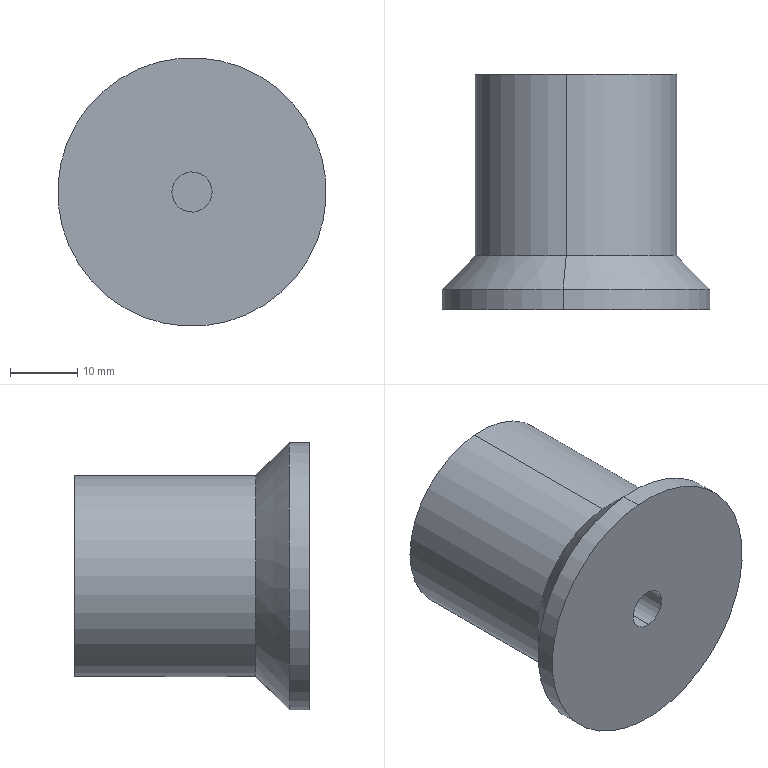Component | SolidWorks | AdjustmentWheel-1 | 1 solid | 13 faces | box 40 x 35 x 40 mm | volume 26932 mm3 | cylinder 8 | plane 3 | cone 2 | commonest cylinder face diameters 2.5 x2 6 x2 40 x2 30 x2
build123d program:
from build123d import *

# Parameters (mm, degrees)
SKETCH2_R      = 3
EXTRUDE2_DEPTH = 25


with BuildPart() as part:
    # Sketch1 → Revolve1 (revolve)
    with BuildSketch(Plane.XY, mode=Mode.PRIVATE) as revolve1_sk:
        Polygon((0, 27.517), (15, 27.517), (15, 0.517), (20, -4.483), (20, -7.483), (0, -7.483), align=None)
    revolve(revolve1_sk.sketch.rotate(Axis((0, 0, 0), (0, 1, 0)), 90), axis=Axis((0, 0, 0), (0, 1, 0)))

    # Sketch2 → Extrude2 (cut)
    with BuildSketch(Plane.XZ.offset(7.483)):
        with Locations(Location((0, 0, 0), (0, 0, 270))):
            Circle(SKETCH2_R)
    extrude(amount=-EXTRUDE2_DEPTH, mode=Mode.SUBTRACT)

    # Sketch3 → M3 Tapped Hole1 (revolve, cut)
    with BuildSketch(Plane(origin=(0, 7.517, 0), x_dir=(0, 1, 0), z_dir=(1, 0, 0))):
        Polygon((0, 0), (0, 20.751), (1.25, 20), (1.25, 0), align=None)
    revolve(axis=Axis((0, 7.517, -6.35), (0, 0, 1)), mode=Mode.SUBTRACT)


solid = part.part

# Placed as in the assembly
solid = solid.moved(Location((-214.784, 725.466, -80.5), (-180, 5.539, 180)))
STEP:
#1=CARTESIAN_POINT('',(-8.399,28.808,-3.757));
#2=VERTEX_POINT('',#1);
#3=CARTESIAN_POINT('',(-8.448,28.858,-3.76));
#4=VERTEX_POINT('',#3);
#5=CARTESIAN_POINT('',(-8.399,28.808,-3.757));
#6=CARTESIAN_POINT('',(-8.405,28.808,-3.758));
#7=CARTESIAN_POINT('',(-8.412,28.81,-3.758));
#8=CARTESIAN_POINT('',(-8.424,28.815,-3.759));
#9=CARTESIAN_POINT('',(-8.429,28.818,-3.759));
#10=CARTESIAN_POINT('',(-8.438,28.827,-3.76));
#11=CARTESIAN_POINT('',(-8.442,28.833,-3.76));
#12=CARTESIAN_POINT('',(-8.446,28.842,-3.76));
#13=CARTESIAN_POINT('',(-8.447,28.845,-3.76));
#14=CARTESIAN_POINT('',(-8.448,28.851,-3.76));
#15=CARTESIAN_POINT('',(-8.448,28.854,-3.76));
#16=CARTESIAN_POINT('',(-8.448,28.858,-3.76));
#17=B_SPLINE_CURVE_WITH_KNOTS('',3,(#5,#6,#7,#8,#9,#10,#11,#12,#13,#14,#15,#16),.UNSPECIFIED.,.F.,.F.,(4,2,2,2,2,4),(0.001955,0.002444,0.002933,0.003421,0.003665,0.00391),.UNSPECIFIED.);
#18=EDGE_CURVE('',#2,#4,#17,.T.);
#19=ORIENTED_EDGE('',*,*,#18,.T.);
#20=CARTESIAN_POINT('',(-8.495,28.858,-3.281));
#21=VERTEX_POINT('',#20);
#22=CARTESIAN_POINT('',(-8.505,28.858,-3.174));
#23=DIRECTION('',(-0.09652,0.,0.9953));
#24=VECTOR('',#23,39.37);
#25=LINE('',#22,#24);
#26=EDGE_CURVE('',#4,#21,#25,.T.);
#27=ORIENTED_EDGE('',*,*,#26,.T.);
#28=CARTESIAN_POINT('',(-8.445,28.808,-3.287));
#29=VERTEX_POINT('',#28);
#30=CARTESIAN_POINT('',(-8.445,28.808,-3.287));
#31=CARTESIAN_POINT('',(-8.448,28.808,-3.287));
#32=CARTESIAN_POINT('',(-8.451,28.809,-3.287));
#33=CARTESIAN_POINT('',(-8.458,28.81,-3.287));
#34=CARTESIAN_POINT('',(-8.461,28.811,-3.287));
#35=CARTESIAN_POINT('',(-8.47,28.815,-3.287));
#36=CARTESIAN_POINT('',(-8.475,28.818,-3.286));
#37=CARTESIAN_POINT('',(-8.484,28.827,-3.284));
#38=CARTESIAN_POINT('',(-8.488,28.833,-3.283));
#39=CARTESIAN_POINT('',(-8.493,28.845,-3.281));
#40=CARTESIAN_POINT('',(-8.495,28.851,-3.281));
#41=CARTESIAN_POINT('',(-8.495,28.858,-3.281));
#42=B_SPLINE_CURVE_WITH_KNOTS('',3,(#30,#31,#32,#33,#34,#35,#36,#37,#38,#39,#40,#41),.UNSPECIFIED.,.F.,.F.,(4,2,2,2,2,4),(0.001977,0.002224,0.002471,0.002965,0.003459,0.003953),.UNSPECIFIED.);
#43=EDGE_CURVE('',#29,#21,#42,.T.);
#44=ORIENTED_EDGE('',*,*,#43,.F.);
#45=CARTESIAN_POINT('',(-8.397,28.858,-3.271));
#46=VERTEX_POINT('',#45);
#47=CARTESIAN_POINT('',(-8.397,28.858,-3.271));
#48=CARTESIAN_POINT('',(-8.397,28.854,-3.271));
#49=CARTESIAN_POINT('',(-8.397,28.851,-3.272));
#50=CARTESIAN_POINT('',(-8.398,28.845,-3.272));
#51=CARTESIAN_POINT('',(-8.399,28.842,-3.273));
#52=CARTESIAN_POINT('',(-8.403,28.833,-3.275));
#53=CARTESIAN_POINT('',(-8.406,28.827,-3.276));
#54=CARTESIAN_POINT('',(-8.415,28.818,-3.28));
#55=CARTESIAN_POINT('',(-8.42,28.815,-3.282));
#56=CARTESIAN_POINT('',(-8.432,28.81,-3.285));
#57=CARTESIAN_POINT('',(-8.438,28.808,-3.286));
#58=CARTESIAN_POINT('',(-8.445,28.808,-3.287));
#59=B_SPLINE_CURVE_WITH_KNOTS('',3,(#47,#48,#49,#50,#51,#52,#53,#54,#55,#56,#57,#58),.UNSPECIFIED.,.F.,.F.,(4,2,2,2,2,4),(0.,0.0002472,0.0004943,0.0009887,0.001483,0.001977),.UNSPECIFIED.);
#60=EDGE_CURVE('',#46,#29,#59,.T.);
#61=ORIENTED_EDGE('',*,*,#60,.F.);
#62=CARTESIAN_POINT('',(-8.35,28.858,-3.75));
#63=VERTEX_POINT('',#62);
#64=CARTESIAN_POINT('',(-8.407,28.858,-3.165));
#65=DIRECTION('',(-0.09652,0.,0.9953));
#66=VECTOR('',#65,39.37);
#67=LINE('',#64,#66);
#68=EDGE_CURVE('',#63,#46,#67,.T.);
#69=ORIENTED_EDGE('',*,*,#68,.F.);
#70=CARTESIAN_POINT('',(-8.35,28.858,-3.75));
#71=CARTESIAN_POINT('',(-8.35,28.851,-3.75));
#72=CARTESIAN_POINT('',(-8.352,28.845,-3.751));
#73=CARTESIAN_POINT('',(-8.356,28.833,-3.751));
#74=CARTESIAN_POINT('',(-8.36,28.827,-3.752));
#75=CARTESIAN_POINT('',(-8.369,28.818,-3.753));
#76=CARTESIAN_POINT('',(-8.374,28.815,-3.754));
#77=CARTESIAN_POINT('',(-8.386,28.81,-3.756));
#78=CARTESIAN_POINT('',(-8.393,28.808,-3.756));
#79=CARTESIAN_POINT('',(-8.399,28.808,-3.757));
#80=B_SPLINE_CURVE_WITH_KNOTS('',3,(#70,#71,#72,#73,#74,#75,#76,#77,#78,#79),.UNSPECIFIED.,.F.,.F.,(4,2,2,2,4),(0.,0.0004888,0.0009777,0.001466,0.001955),.UNSPECIFIED.);
#81=EDGE_CURVE('',#63,#2,#80,.T.);
#82=ORIENTED_EDGE('',*,*,#81,.T.);
#83=EDGE_LOOP('',(#19,#27,#44,#61,#69,#82));
#84=FACE_OUTER_BOUND('',#83,.T.);
#85=CARTESIAN_POINT('',(-8.456,28.858,-3.169));
#86=DIRECTION('',(-0.09652,0.,0.9953));
#87=DIRECTION('',(0.9953,0.,0.09652));
#88=AXIS2_PLACEMENT_3D('',#85,#86,#87);
#89=CYLINDRICAL_SURFACE('',#88,0.04921);
#90=ADVANCED_FACE('',(#84),#89,.F.);
#91=CARTESIAN_POINT('',(-8.445,29.251,-3.287));
#92=VERTEX_POINT('',#91);
#93=CARTESIAN_POINT('',(-8.467,29.251,-3.052));
#94=VERTEX_POINT('',#93);
#95=CARTESIAN_POINT('',(-8.456,29.251,-3.169));
#96=DIRECTION('',(0.,-1.,0.));
#97=DIRECTION('',(-0.09652,0.,0.9953));
#98=AXIS2_PLACEMENT_3D('',#95,#96,#97);
#99=CIRCLE('',#98,0.1181);
#100=EDGE_CURVE('',#92,#94,#99,.T.);
#101=ORIENTED_EDGE('',*,*,#100,.F.);
#102=CARTESIAN_POINT('',(-8.445,28.907,-3.287));
#103=VERTEX_POINT('',#102);
#104=CARTESIAN_POINT('',(-8.445,29.251,-3.287));
#105=DIRECTION('',(0.,-1.,0.));
#106=VECTOR('',#105,39.37);
#107=LINE('',#104,#106);
#108=EDGE_CURVE('',#92,#103,#107,.T.);
#109=ORIENTED_EDGE('',*,*,#108,.T.);
#110=CARTESIAN_POINT('',(-8.445,28.907,-3.287));
#111=CARTESIAN_POINT('',(-8.438,28.907,-3.286));
#112=CARTESIAN_POINT('',(-8.432,28.906,-3.285));
#113=CARTESIAN_POINT('',(-8.42,28.901,-3.282));
#114=CARTESIAN_POINT('',(-8.415,28.897,-3.28));
#115=CARTESIAN_POINT('',(-8.406,28.888,-3.276));
#116=CARTESIAN_POINT('',(-8.403,28.883,-3.275));
#117=CARTESIAN_POINT('',(-8.398,28.871,-3.272));
#118=CARTESIAN_POINT('',(-8.397,28.864,-3.271));
#119=CARTESIAN_POINT('',(-8.397,28.858,-3.271));
#120=B_SPLINE_CURVE_WITH_KNOTS('',3,(#110,#111,#112,#113,#114,#115,#116,#117,#118,#119),.UNSPECIFIED.,.F.,.F.,(4,2,2,2,4),(0.005929,0.006423,0.006916,0.00741,0.007904),.UNSPECIFIED.);
#121=EDGE_CURVE('',#103,#46,#120,.T.);
#122=ORIENTED_EDGE('',*,*,#121,.T.);
#123=ORIENTED_EDGE('',*,*,#60,.T.);
#124=CARTESIAN_POINT('',(-8.445,28.267,-3.287));
#125=VERTEX_POINT('',#124);
#126=CARTESIAN_POINT('',(-8.445,29.251,-3.287));
#127=DIRECTION('',(0.,-1.,0.));
#128=VECTOR('',#127,39.37);
#129=LINE('',#126,#128);
#130=EDGE_CURVE('',#29,#125,#129,.T.);
#131=ORIENTED_EDGE('',*,*,#130,.T.);
#132=CARTESIAN_POINT('',(-8.467,28.267,-3.052));
#133=VERTEX_POINT('',#132);
#134=CARTESIAN_POINT('',(-8.456,28.267,-3.169));
#135=DIRECTION('',(0.,-1.,0.));
#136=DIRECTION('',(-0.09652,0.,0.9953));
#137=AXIS2_PLACEMENT_3D('',#134,#135,#136);
#138=CIRCLE('',#137,0.1181);
#139=EDGE_CURVE('',#125,#133,#138,.T.);
#140=ORIENTED_EDGE('',*,*,#139,.T.);
#141=CARTESIAN_POINT('',(-8.467,29.251,-3.052));
#142=DIRECTION('',(0.,-1.,0.));
#143=VECTOR('',#142,39.37);
#144=LINE('',#141,#143);
#145=EDGE_CURVE('',#94,#133,#144,.T.);
#146=ORIENTED_EDGE('',*,*,#145,.F.);
#147=EDGE_LOOP('',(#101,#109,#122,#123,#131,#140,#146));
#148=FACE_OUTER_BOUND('',#147,.T.);
#149=CARTESIAN_POINT('',(-8.456,29.251,-3.169));
#150=DIRECTION('',(0.,-1.,0.));
#151=DIRECTION('',(-0.09652,0.,0.9953));
#152=AXIS2_PLACEMENT_3D('',#149,#150,#151);
#153=CYLINDRICAL_SURFACE('',#152,0.1181);
#154=ADVANCED_FACE('',(#148),#153,.F.);
#155=CARTESIAN_POINT('',(-8.532,28.385,-2.386));
#156=VERTEX_POINT('',#155);
#157=CARTESIAN_POINT('',(-8.38,28.385,-3.953));
#158=VERTEX_POINT('',#157);
#159=CARTESIAN_POINT('',(-8.456,28.385,-3.169));
#160=DIRECTION('',(0.,-1.,0.));
#161=DIRECTION('',(-0.09652,0.,0.9953));
#162=AXIS2_PLACEMENT_3D('',#159,#160,#161);
#163=CIRCLE('',#162,0.7874);
#164=EDGE_CURVE('',#156,#158,#163,.T.);
#165=ORIENTED_EDGE('',*,*,#164,.T.);
#166=CARTESIAN_POINT('',(-8.38,28.267,-3.953));
#167=VERTEX_POINT('',#166);
#168=CARTESIAN_POINT('',(-8.38,28.562,-3.953));
#169=DIRECTION('',(0.,-1.,0.));
#170=VECTOR('',#169,39.37);
#171=LINE('',#168,#170);
#172=EDGE_CURVE('',#158,#167,#171,.T.);
#173=ORIENTED_EDGE('',*,*,#172,.T.);
#174=CARTESIAN_POINT('',(-8.532,28.267,-2.386));
#175=VERTEX_POINT('',#174);
#176=CARTESIAN_POINT('',(-8.456,28.267,-3.169));
#177=DIRECTION('',(0.,-1.,0.));
#178=DIRECTION('',(-0.09652,0.,0.9953));
#179=AXIS2_PLACEMENT_3D('',#176,#177,#178);
#180=CIRCLE('',#179,0.7874);
#181=EDGE_CURVE('',#175,#167,#180,.T.);
#182=ORIENTED_EDGE('',*,*,#181,.F.);
#183=CARTESIAN_POINT('',(-8.532,28.562,-2.386));
#184=DIRECTION('',(0.,-1.,0.));
#185=VECTOR('',#184,39.37);
#186=LINE('',#183,#185);
#187=EDGE_CURVE('',#156,#175,#186,.T.);
#188=ORIENTED_EDGE('',*,*,#187,.F.);
#189=EDGE_LOOP('',(#165,#173,#182,#188));
#190=FACE_OUTER_BOUND('',#189,.T.);
#191=CARTESIAN_POINT('',(-8.456,28.562,-3.169));
#192=DIRECTION('',(0.,-1.,0.));
#193=DIRECTION('',(-0.09652,0.,0.9953));
#194=AXIS2_PLACEMENT_3D('',#191,#192,#193);
#195=CYLINDRICAL_SURFACE('',#194,0.7874);
#196=ADVANCED_FACE('',(#190),#195,.T.);
#197=CARTESIAN_POINT('',(-8.513,28.582,-2.581));
#198=VERTEX_POINT('',#197);
#199=CARTESIAN_POINT('',(-8.399,28.582,-3.757));
#200=VERTEX_POINT('',#199);
#201=CARTESIAN_POINT('',(-8.456,28.582,-3.169));
#202=DIRECTION('',(0.,-1.,0.));
#203=DIRECTION('',(-0.09652,0.,0.9953));
#204=AXIS2_PLACEMENT_3D('',#201,#202,#203);
#205=CIRCLE('',#204,0.5906);
#206=EDGE_CURVE('',#198,#200,#205,.T.);
#207=ORIENTED_EDGE('',*,*,#206,.T.);
#208=CARTESIAN_POINT('',(-8.38,28.385,-3.953));
#209=DIRECTION('',(0.06825,-0.7071,-0.7038));
#210=VECTOR('',#209,39.37);
#211=LINE('',#208,#210);
#212=EDGE_CURVE('',#200,#158,#211,.T.);
#213=ORIENTED_EDGE('',*,*,#212,.T.);
#214=ORIENTED_EDGE('',*,*,#164,.F.);
#215=CARTESIAN_POINT('',(-8.532,28.385,-2.386));
#216=DIRECTION('',(-0.06825,-0.7071,0.7038));
#217=VECTOR('',#216,39.37);
#218=LINE('',#215,#217);
#219=EDGE_CURVE('',#198,#156,#218,.T.);
#220=ORIENTED_EDGE('',*,*,#219,.F.);
#221=EDGE_LOOP('',(#207,#213,#214,#220));
#222=FACE_OUTER_BOUND('',#221,.T.);
#223=CARTESIAN_POINT('',(-8.456,28.385,-3.169));
#224=DIRECTION('',(0.,-1.,0.));
#225=DIRECTION('',(-0.09652,0.,0.9953));
#226=AXIS2_PLACEMENT_3D('',#223,#224,#225);
#227=CONICAL_SURFACE('',#226,0.7874,0.7854);
#228=ADVANCED_FACE('',(#222),#227,.T.);
#229=CARTESIAN_POINT('',(-8.513,29.645,-2.581));
#230=VERTEX_POINT('',#229);
#231=CARTESIAN_POINT('',(-8.399,29.645,-3.757));
#232=VERTEX_POINT('',#231);
#233=CARTESIAN_POINT('',(-8.456,29.645,-3.169));
#234=DIRECTION('',(0.,-1.,0.));
#235=DIRECTION('',(-0.09652,0.,0.9953));
#236=AXIS2_PLACEMENT_3D('',#233,#234,#235);
#237=CIRCLE('',#236,0.5906);
#238=EDGE_CURVE('',#230,#232,#237,.T.);
#239=ORIENTED_EDGE('',*,*,#238,.T.);
#240=CARTESIAN_POINT('',(-8.399,28.907,-3.757));
#241=VERTEX_POINT('',#240);
#242=CARTESIAN_POINT('',(-8.399,28.562,-3.757));
#243=DIRECTION('',(0.,-1.,0.));
#244=VECTOR('',#243,39.37);
#245=LINE('',#242,#244);
#246=EDGE_CURVE('',#232,#241,#245,.T.);
#247=ORIENTED_EDGE('',*,*,#246,.T.);
#248=CARTESIAN_POINT('',(-8.448,28.858,-3.76));
#249=CARTESIAN_POINT('',(-8.448,28.864,-3.76));
#250=CARTESIAN_POINT('',(-8.447,28.871,-3.76));
#251=CARTESIAN_POINT('',(-8.442,28.882,-3.76));
#252=CARTESIAN_POINT('',(-8.438,28.888,-3.76));
#253=CARTESIAN_POINT('',(-8.429,28.897,-3.759));
#254=CARTESIAN_POINT('',(-8.424,28.901,-3.759));
#255=CARTESIAN_POINT('',(-8.412,28.906,-3.758));
#256=CARTESIAN_POINT('',(-8.406,28.907,-3.758));
#257=CARTESIAN_POINT('',(-8.399,28.907,-3.757));
#258=B_SPLINE_CURVE_WITH_KNOTS('',3,(#248,#249,#250,#251,#252,#253,#254,#255,#256,#257),.UNSPECIFIED.,.F.,.F.,(4,2,2,2,4),(0.00391,0.004399,0.004887,0.005376,0.005865),.UNSPECIFIED.);
#259=EDGE_CURVE('',#4,#241,#258,.T.);
#260=ORIENTED_EDGE('',*,*,#259,.F.);
#261=ORIENTED_EDGE('',*,*,#18,.F.);
#262=CARTESIAN_POINT('',(-8.399,28.562,-3.757));
#263=DIRECTION('',(0.,-1.,0.));
#264=VECTOR('',#263,39.37);
#265=LINE('',#262,#264);
#266=EDGE_CURVE('',#2,#200,#265,.T.);
#267=ORIENTED_EDGE('',*,*,#266,.T.);
#268=ORIENTED_EDGE('',*,*,#206,.F.);
#269=CARTESIAN_POINT('',(-8.513,28.562,-2.581));
#270=DIRECTION('',(0.,-1.,0.));
#271=VECTOR('',#270,39.37);
#272=LINE('',#269,#271);
#273=EDGE_CURVE('',#230,#198,#272,.T.);
#274=ORIENTED_EDGE('',*,*,#273,.F.);
#275=EDGE_LOOP('',(#239,#247,#260,#261,#267,#268,#274));
#276=FACE_OUTER_BOUND('',#275,.T.);
#277=CARTESIAN_POINT('',(-8.456,28.562,-3.169));
#278=DIRECTION('',(0.,-1.,0.));
#279=DIRECTION('',(-0.09652,0.,0.9953));
#280=AXIS2_PLACEMENT_3D('',#277,#278,#279);
#281=CYLINDRICAL_SURFACE('',#280,0.5906);
#282=ADVANCED_FACE('',(#276),#281,.T.);
#283=ORIENTED_EDGE('',*,*,#238,.F.);
#284=CARTESIAN_POINT('',(-8.456,29.645,-3.169));
#285=DIRECTION('',(0.,-1.,0.));
#286=DIRECTION('',(-0.09652,0.,0.9953));
#287=AXIS2_PLACEMENT_3D('',#284,#285,#286);
#288=CIRCLE('',#287,0.5906);
#289=EDGE_CURVE('',#232,#230,#288,.T.);
#290=ORIENTED_EDGE('',*,*,#289,.F.);
#291=EDGE_LOOP('',(#283,#290));
#292=FACE_OUTER_BOUND('',#291,.T.);
#293=CARTESIAN_POINT('',(-8.456,29.645,-3.169));
#294=DIRECTION('',(0.,1.,0.));
#295=DIRECTION('',(0.09652,0.,-0.9953));
#296=AXIS2_PLACEMENT_3D('',#293,#294,#295);
#297=PLANE('',#296);
#298=ADVANCED_FACE('',(#292),#297,.T.);
#299=ORIENTED_EDGE('',*,*,#246,.F.);
#300=ORIENTED_EDGE('',*,*,#289,.T.);
#301=ORIENTED_EDGE('',*,*,#273,.T.);
#302=CARTESIAN_POINT('',(-8.456,28.582,-3.169));
#303=DIRECTION('',(0.,-1.,0.));
#304=DIRECTION('',(-0.09652,0.,0.9953));
#305=AXIS2_PLACEMENT_3D('',#302,#303,#304);
#306=CIRCLE('',#305,0.5906);
#307=EDGE_CURVE('',#200,#198,#306,.T.);
#308=ORIENTED_EDGE('',*,*,#307,.F.);
#309=ORIENTED_EDGE('',*,*,#266,.F.);
#310=ORIENTED_EDGE('',*,*,#81,.F.);
#311=CARTESIAN_POINT('',(-8.399,28.907,-3.757));
#312=CARTESIAN_POINT('',(-8.393,28.907,-3.756));
#313=CARTESIAN_POINT('',(-8.386,28.906,-3.756));
#314=CARTESIAN_POINT('',(-8.377,28.902,-3.755));
#315=CARTESIAN_POINT('',(-8.375,28.9,-3.754));
#316=CARTESIAN_POINT('',(-8.369,28.897,-3.753));
#317=CARTESIAN_POINT('',(-8.367,28.895,-3.753));
#318=CARTESIAN_POINT('',(-8.36,28.888,-3.752));
#319=CARTESIAN_POINT('',(-8.356,28.882,-3.751));
#320=CARTESIAN_POINT('',(-8.352,28.871,-3.751));
#321=CARTESIAN_POINT('',(-8.35,28.864,-3.75));
#322=CARTESIAN_POINT('',(-8.35,28.858,-3.75));
#323=B_SPLINE_CURVE_WITH_KNOTS('',3,(#311,#312,#313,#314,#315,#316,#317,#318,#319,#320,#321,#322),.UNSPECIFIED.,.F.,.F.,(4,2,2,2,2,4),(0.005865,0.006354,0.006598,0.006842,0.00733,0.007819),.UNSPECIFIED.);
#324=EDGE_CURVE('',#241,#63,#323,.T.);
#325=ORIENTED_EDGE('',*,*,#324,.F.);
#326=EDGE_LOOP('',(#299,#300,#301,#308,#309,#310,#325));
#327=FACE_OUTER_BOUND('',#326,.T.);
#328=CARTESIAN_POINT('',(-8.456,28.562,-3.169));
#329=DIRECTION('',(0.,-1.,0.));
#330=DIRECTION('',(-0.09652,0.,0.9953));
#331=AXIS2_PLACEMENT_3D('',#328,#329,#330);
#332=CYLINDRICAL_SURFACE('',#331,0.5906);
#333=ADVANCED_FACE('',(#327),#332,.T.);
#334=ORIENTED_EDGE('',*,*,#212,.F.);
#335=ORIENTED_EDGE('',*,*,#307,.T.);
#336=ORIENTED_EDGE('',*,*,#219,.T.);
#337=CARTESIAN_POINT('',(-8.456,28.385,-3.169));
#338=DIRECTION('',(0.,-1.,0.));
#339=DIRECTION('',(-0.09652,0.,0.9953));
#340=AXIS2_PLACEMENT_3D('',#337,#338,#339);
#341=CIRCLE('',#340,0.7874);
#342=EDGE_CURVE('',#158,#156,#341,.T.);
#343=ORIENTED_EDGE('',*,*,#342,.F.);
#344=EDGE_LOOP('',(#334,#335,#336,#343));
#345=FACE_OUTER_BOUND('',#344,.T.);
#346=CARTESIAN_POINT('',(-8.456,28.385,-3.169));
#347=DIRECTION('',(0.,-1.,0.));
#348=DIRECTION('',(-0.09652,0.,0.9953));
#349=AXIS2_PLACEMENT_3D('',#346,#347,#348);
#350=CONICAL_SURFACE('',#349,0.7874,0.7854);
#351=ADVANCED_FACE('',(#345),#350,.T.);
#352=ORIENTED_EDGE('',*,*,#172,.F.);
#353=ORIENTED_EDGE('',*,*,#342,.T.);
#354=ORIENTED_EDGE('',*,*,#187,.T.);
#355=CARTESIAN_POINT('',(-8.456,28.267,-3.169));
#356=DIRECTION('',(0.,-1.,0.));
#357=DIRECTION('',(-0.09652,0.,0.9953));
#358=AXIS2_PLACEMENT_3D('',#355,#356,#357);
#359=CIRCLE('',#358,0.7874);
#360=EDGE_CURVE('',#167,#175,#359,.T.);
#361=ORIENTED_EDGE('',*,*,#360,.F.);
#362=EDGE_LOOP('',(#352,#353,#354,#361));
#363=FACE_OUTER_BOUND('',#362,.T.);
#364=CARTESIAN_POINT('',(-8.456,28.562,-3.169));
#365=DIRECTION('',(0.,-1.,0.));
#366=DIRECTION('',(-0.09652,0.,0.9953));
#367=AXIS2_PLACEMENT_3D('',#364,#365,#366);
#368=CYLINDRICAL_SURFACE('',#367,0.7874);
#369=ADVANCED_FACE('',(#363),#368,.T.);
#370=CARTESIAN_POINT('',(-8.456,28.267,-3.169));
#371=DIRECTION('',(0.,-1.,0.));
#372=DIRECTION('',(-0.09652,0.,0.9953));
#373=AXIS2_PLACEMENT_3D('',#370,#371,#372);
#374=CIRCLE('',#373,0.1181);
#375=EDGE_CURVE('',#133,#125,#374,.T.);
#376=ORIENTED_EDGE('',*,*,#375,.F.);
#377=ORIENTED_EDGE('',*,*,#139,.F.);
#378=EDGE_LOOP('',(#376,#377));
#379=FACE_BOUND('',#378,.T.);
#380=ORIENTED_EDGE('',*,*,#181,.T.);
#381=ORIENTED_EDGE('',*,*,#360,.T.);
#382=EDGE_LOOP('',(#380,#381));
#383=FACE_OUTER_BOUND('',#382,.T.);
#384=CARTESIAN_POINT('',(-9.24,28.267,-3.245));
#385=DIRECTION('',(0.,-1.,0.));
#386=DIRECTION('',(-0.09652,0.,0.9953));
#387=AXIS2_PLACEMENT_3D('',#384,#385,#386);
#388=PLANE('',#387);
#389=ADVANCED_FACE('',(#379,#383),#388,.T.);
#390=ORIENTED_EDGE('',*,*,#108,.F.);
#391=CARTESIAN_POINT('',(-8.456,29.251,-3.169));
#392=DIRECTION('',(0.,-1.,0.));
#393=DIRECTION('',(-0.09652,0.,0.9953));
#394=AXIS2_PLACEMENT_3D('',#391,#392,#393);
#395=CIRCLE('',#394,0.1181);
#396=EDGE_CURVE('',#94,#92,#395,.T.);
#397=ORIENTED_EDGE('',*,*,#396,.F.);
#398=ORIENTED_EDGE('',*,*,#145,.T.);
#399=ORIENTED_EDGE('',*,*,#375,.T.);
#400=ORIENTED_EDGE('',*,*,#130,.F.);
#401=ORIENTED_EDGE('',*,*,#43,.T.);
#402=CARTESIAN_POINT('',(-8.495,28.858,-3.281));
#403=CARTESIAN_POINT('',(-8.495,28.864,-3.281));
#404=CARTESIAN_POINT('',(-8.493,28.871,-3.281));
#405=CARTESIAN_POINT('',(-8.488,28.883,-3.283));
#406=CARTESIAN_POINT('',(-8.484,28.888,-3.284));
#407=CARTESIAN_POINT('',(-8.477,28.895,-3.285));
#408=CARTESIAN_POINT('',(-8.475,28.897,-3.286));
#409=CARTESIAN_POINT('',(-8.47,28.9,-3.287));
#410=CARTESIAN_POINT('',(-8.467,28.902,-3.287));
#411=CARTESIAN_POINT('',(-8.461,28.904,-3.287));
#412=CARTESIAN_POINT('',(-8.458,28.905,-3.287));
#413=CARTESIAN_POINT('',(-8.451,28.906,-3.287));
#414=CARTESIAN_POINT('',(-8.448,28.907,-3.287));
#415=CARTESIAN_POINT('',(-8.445,28.907,-3.287));
#416=B_SPLINE_CURVE_WITH_KNOTS('',3,(#402,#403,#404,#405,#406,#407,#408,#409,#410,#411,#412,#413,#414,#415),.UNSPECIFIED.,.F.,.F.,(4,2,2,2,2,2,4),(0.003953,0.004447,0.004941,0.005188,0.005435,0.005682,0.005929),.UNSPECIFIED.);
#417=EDGE_CURVE('',#21,#103,#416,.T.);
#418=ORIENTED_EDGE('',*,*,#417,.T.);
#419=EDGE_LOOP('',(#390,#397,#398,#399,#400,#401,#418));
#420=FACE_OUTER_BOUND('',#419,.T.);
#421=CARTESIAN_POINT('',(-8.456,29.251,-3.169));
#422=DIRECTION('',(0.,-1.,0.));
#423=DIRECTION('',(-0.09652,0.,0.9953));
#424=AXIS2_PLACEMENT_3D('',#421,#422,#423);
#425=CYLINDRICAL_SURFACE('',#424,0.1181);
#426=ADVANCED_FACE('',(#420),#425,.F.);
#427=ORIENTED_EDGE('',*,*,#396,.T.);
#428=ORIENTED_EDGE('',*,*,#100,.T.);
#429=EDGE_LOOP('',(#427,#428));
#430=FACE_OUTER_BOUND('',#429,.T.);
#431=CARTESIAN_POINT('',(-8.456,29.251,-3.169));
#432=DIRECTION('',(0.,-1.,0.));
#433=DIRECTION('',(-0.09652,0.,0.9953));
#434=AXIS2_PLACEMENT_3D('',#431,#432,#433);
#435=PLANE('',#434);
#436=ADVANCED_FACE('',(#430),#435,.T.);
#437=ORIENTED_EDGE('',*,*,#26,.F.);
#438=ORIENTED_EDGE('',*,*,#259,.T.);
#439=ORIENTED_EDGE('',*,*,#324,.T.);
#440=ORIENTED_EDGE('',*,*,#68,.T.);
#441=ORIENTED_EDGE('',*,*,#121,.F.);
#442=ORIENTED_EDGE('',*,*,#417,.F.);
#443=EDGE_LOOP('',(#437,#438,#439,#440,#441,#442));
#444=FACE_OUTER_BOUND('',#443,.T.);
#445=CARTESIAN_POINT('',(-8.456,28.858,-3.169));
#446=DIRECTION('',(-0.09652,0.,0.9953));
#447=DIRECTION('',(0.9953,0.,0.09652));
#448=AXIS2_PLACEMENT_3D('',#445,#446,#447);
#449=CYLINDRICAL_SURFACE('',#448,0.04921);
#450=ADVANCED_FACE('',(#444),#449,.F.);
#451=CLOSED_SHELL('',(#90,#154,#196,#228,#282,#298,#333,#351,#369,#389,#426,#436,#450));
#452=MANIFOLD_SOLID_BREP('',#451);
#453=CARTESIAN_POINT('',(0.,0.,0.));
#454=DIRECTION('',(0.,0.,1.));
#455=DIRECTION('',(1.,0.,0.));
#456=AXIS2_PLACEMENT_3D('',#453,#454,#455);
#457=(LENGTH_UNIT()NAMED_UNIT(*)SI_UNIT($,.METRE.));
#458=LENGTH_MEASURE_WITH_UNIT(LENGTH_MEASURE(0.0254),#457);
#459=DIMENSIONAL_EXPONENTS(1.,0.,0.,0.,0.,0.,0.);
#460=(CONVERSION_BASED_UNIT('',#458)LENGTH_UNIT()NAMED_UNIT(#459));
#461=UNCERTAINTY_MEASURE_WITH_UNIT(LENGTH_MEASURE(0.00001),#460,'','');
#462=(NAMED_UNIT(*)PLANE_ANGLE_UNIT()SI_UNIT($,.RADIAN.));
#463=(NAMED_UNIT(*)SI_UNIT($,.STERADIAN.)SOLID_ANGLE_UNIT());
#464=(GEOMETRIC_REPRESENTATION_CONTEXT(3)GLOBAL_UNCERTAINTY_ASSIGNED_CONTEXT((#461))GLOBAL_UNIT_ASSIGNED_CONTEXT((#460,#462,#463))REPRESENTATION_CONTEXT('',''));
#465=ADVANCED_BREP_SHAPE_REPRESENTATION('',(#452,#456),#464);
#466=COLOUR_RGB('',0.7922,0.8196,0.9333);
#467=FILL_AREA_STYLE_COLOUR('',#466);
#468=FILL_AREA_STYLE('',(#467));
#469=SURFACE_STYLE_FILL_AREA(#468);
#470=SURFACE_SIDE_STYLE('',(#469));
#471=SURFACE_STYLE_USAGE(.BOTH.,#470);
#472=PRESENTATION_STYLE_ASSIGNMENT((#471));
#473=STYLED_ITEM('',(#472),#452);
#474=(LENGTH_UNIT()NAMED_UNIT(*)SI_UNIT($,.METRE.));
#475=LENGTH_MEASURE_WITH_UNIT(LENGTH_MEASURE(0.0254),#474);
#476=DIMENSIONAL_EXPONENTS(1.,0.,0.,0.,0.,0.,0.);
#477=(CONVERSION_BASED_UNIT('',#475)LENGTH_UNIT()NAMED_UNIT(#476));
#478=UNCERTAINTY_MEASURE_WITH_UNIT(LENGTH_MEASURE(0.00001),#477,'','');
#479=(NAMED_UNIT(*)PLANE_ANGLE_UNIT()SI_UNIT($,.RADIAN.));
#480=(NAMED_UNIT(*)SI_UNIT($,.STERADIAN.)SOLID_ANGLE_UNIT());
#481=(GEOMETRIC_REPRESENTATION_CONTEXT(3)GLOBAL_UNCERTAINTY_ASSIGNED_CONTEXT((#478))GLOBAL_UNIT_ASSIGNED_CONTEXT((#477,#479,#480))REPRESENTATION_CONTEXT('',''));
#482=MECHANICAL_DESIGN_GEOMETRIC_PRESENTATION_REPRESENTATION('',(#473),#481);
#483=PRESENTATION_LAYER_ASSIGNMENT('','',(#473));